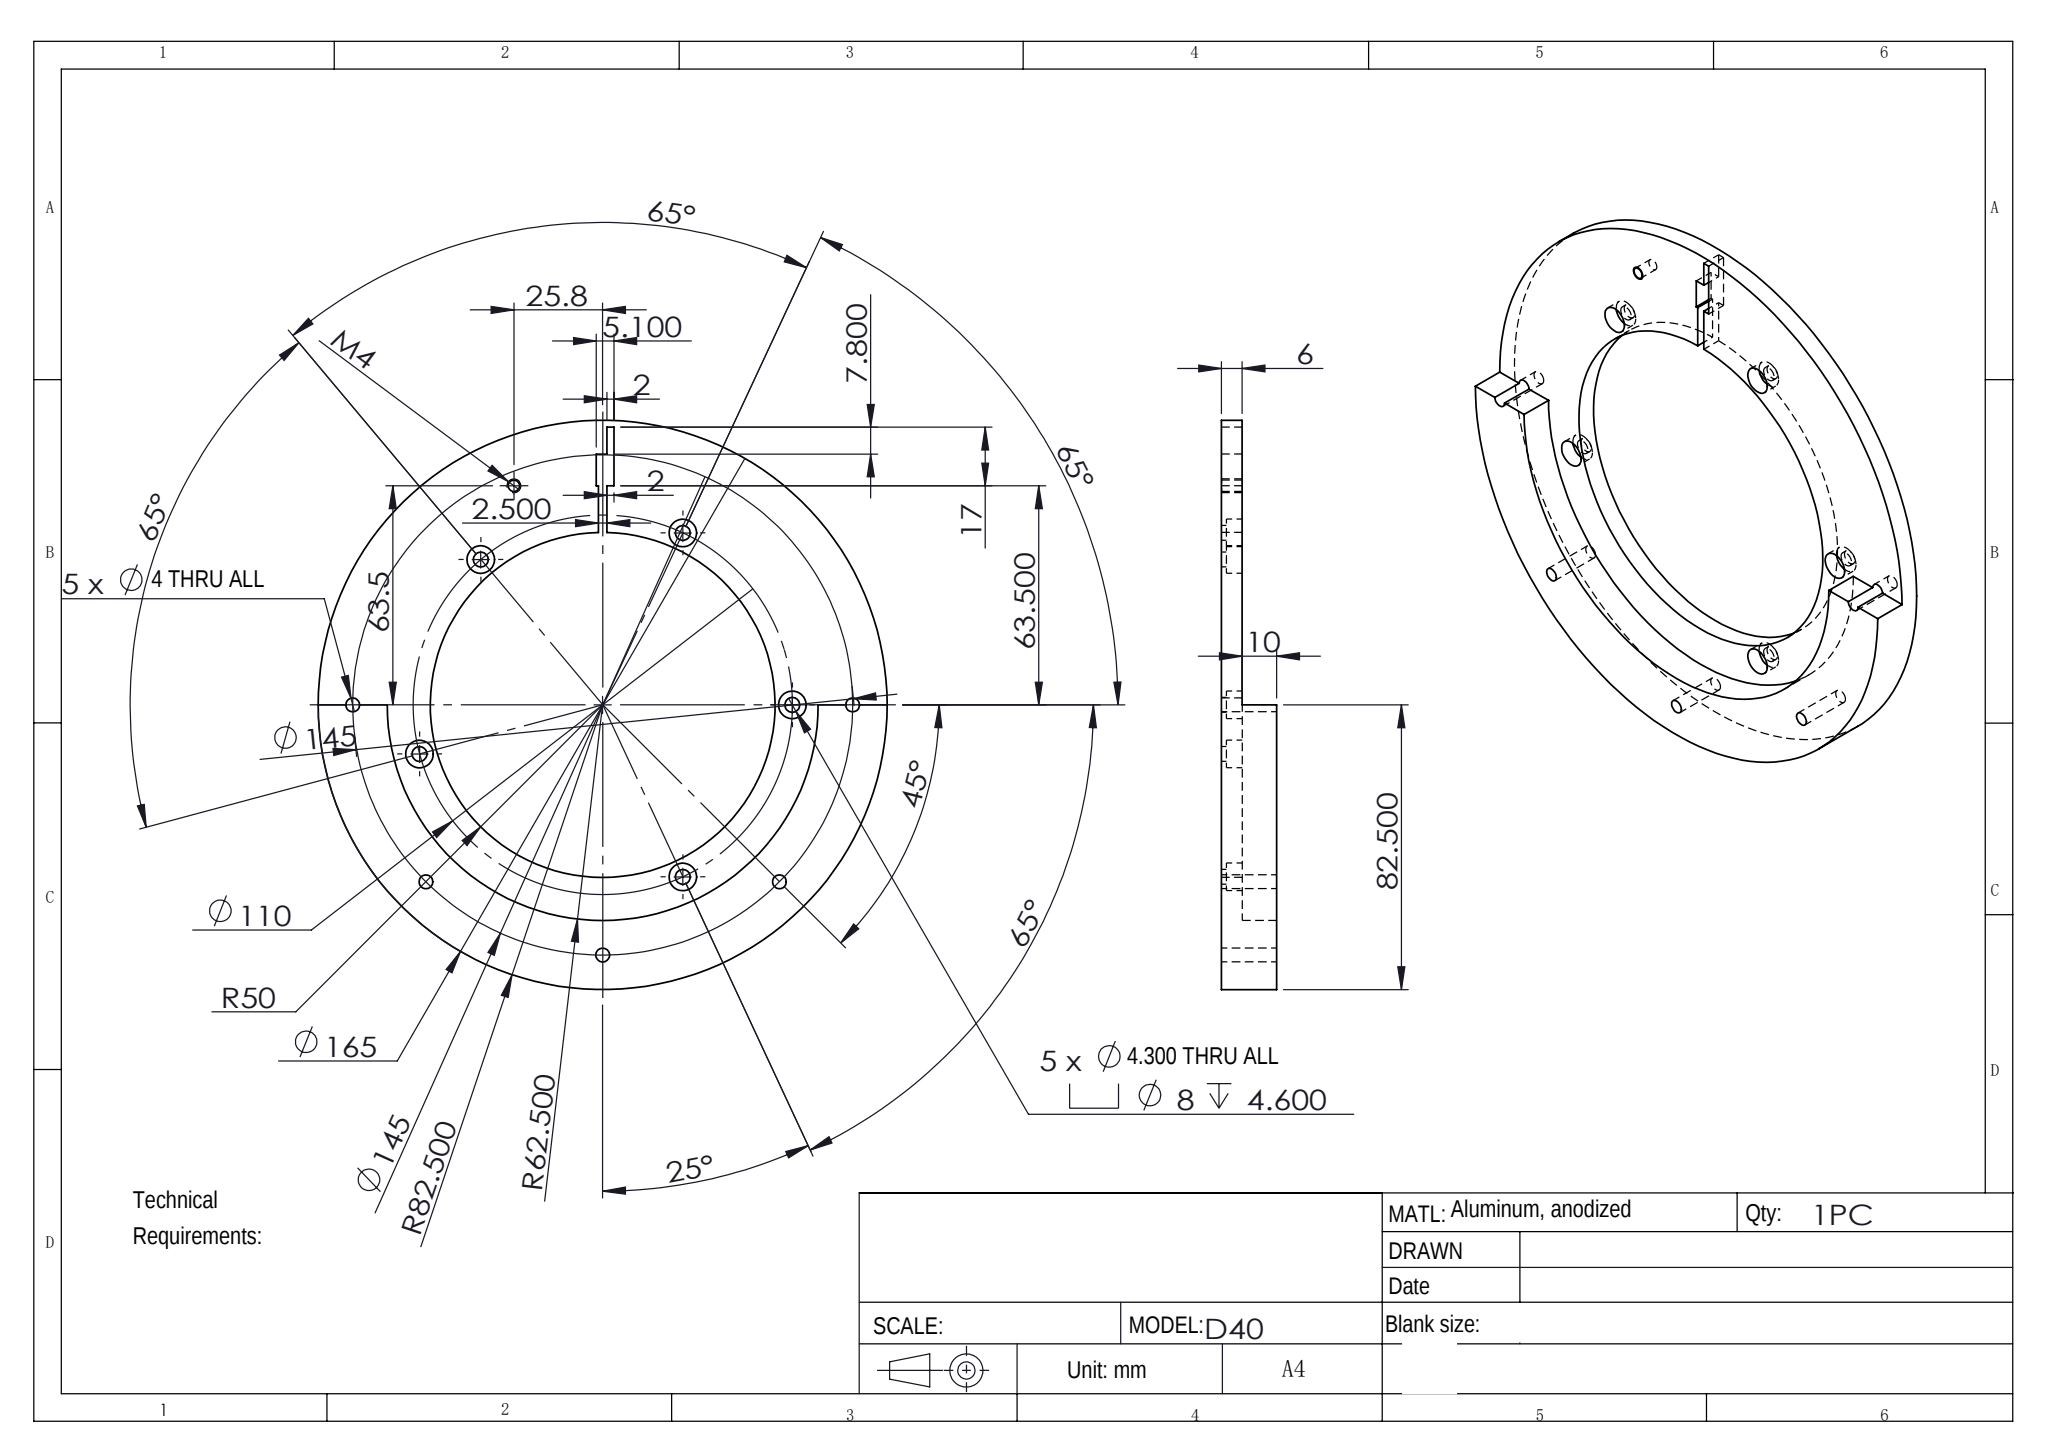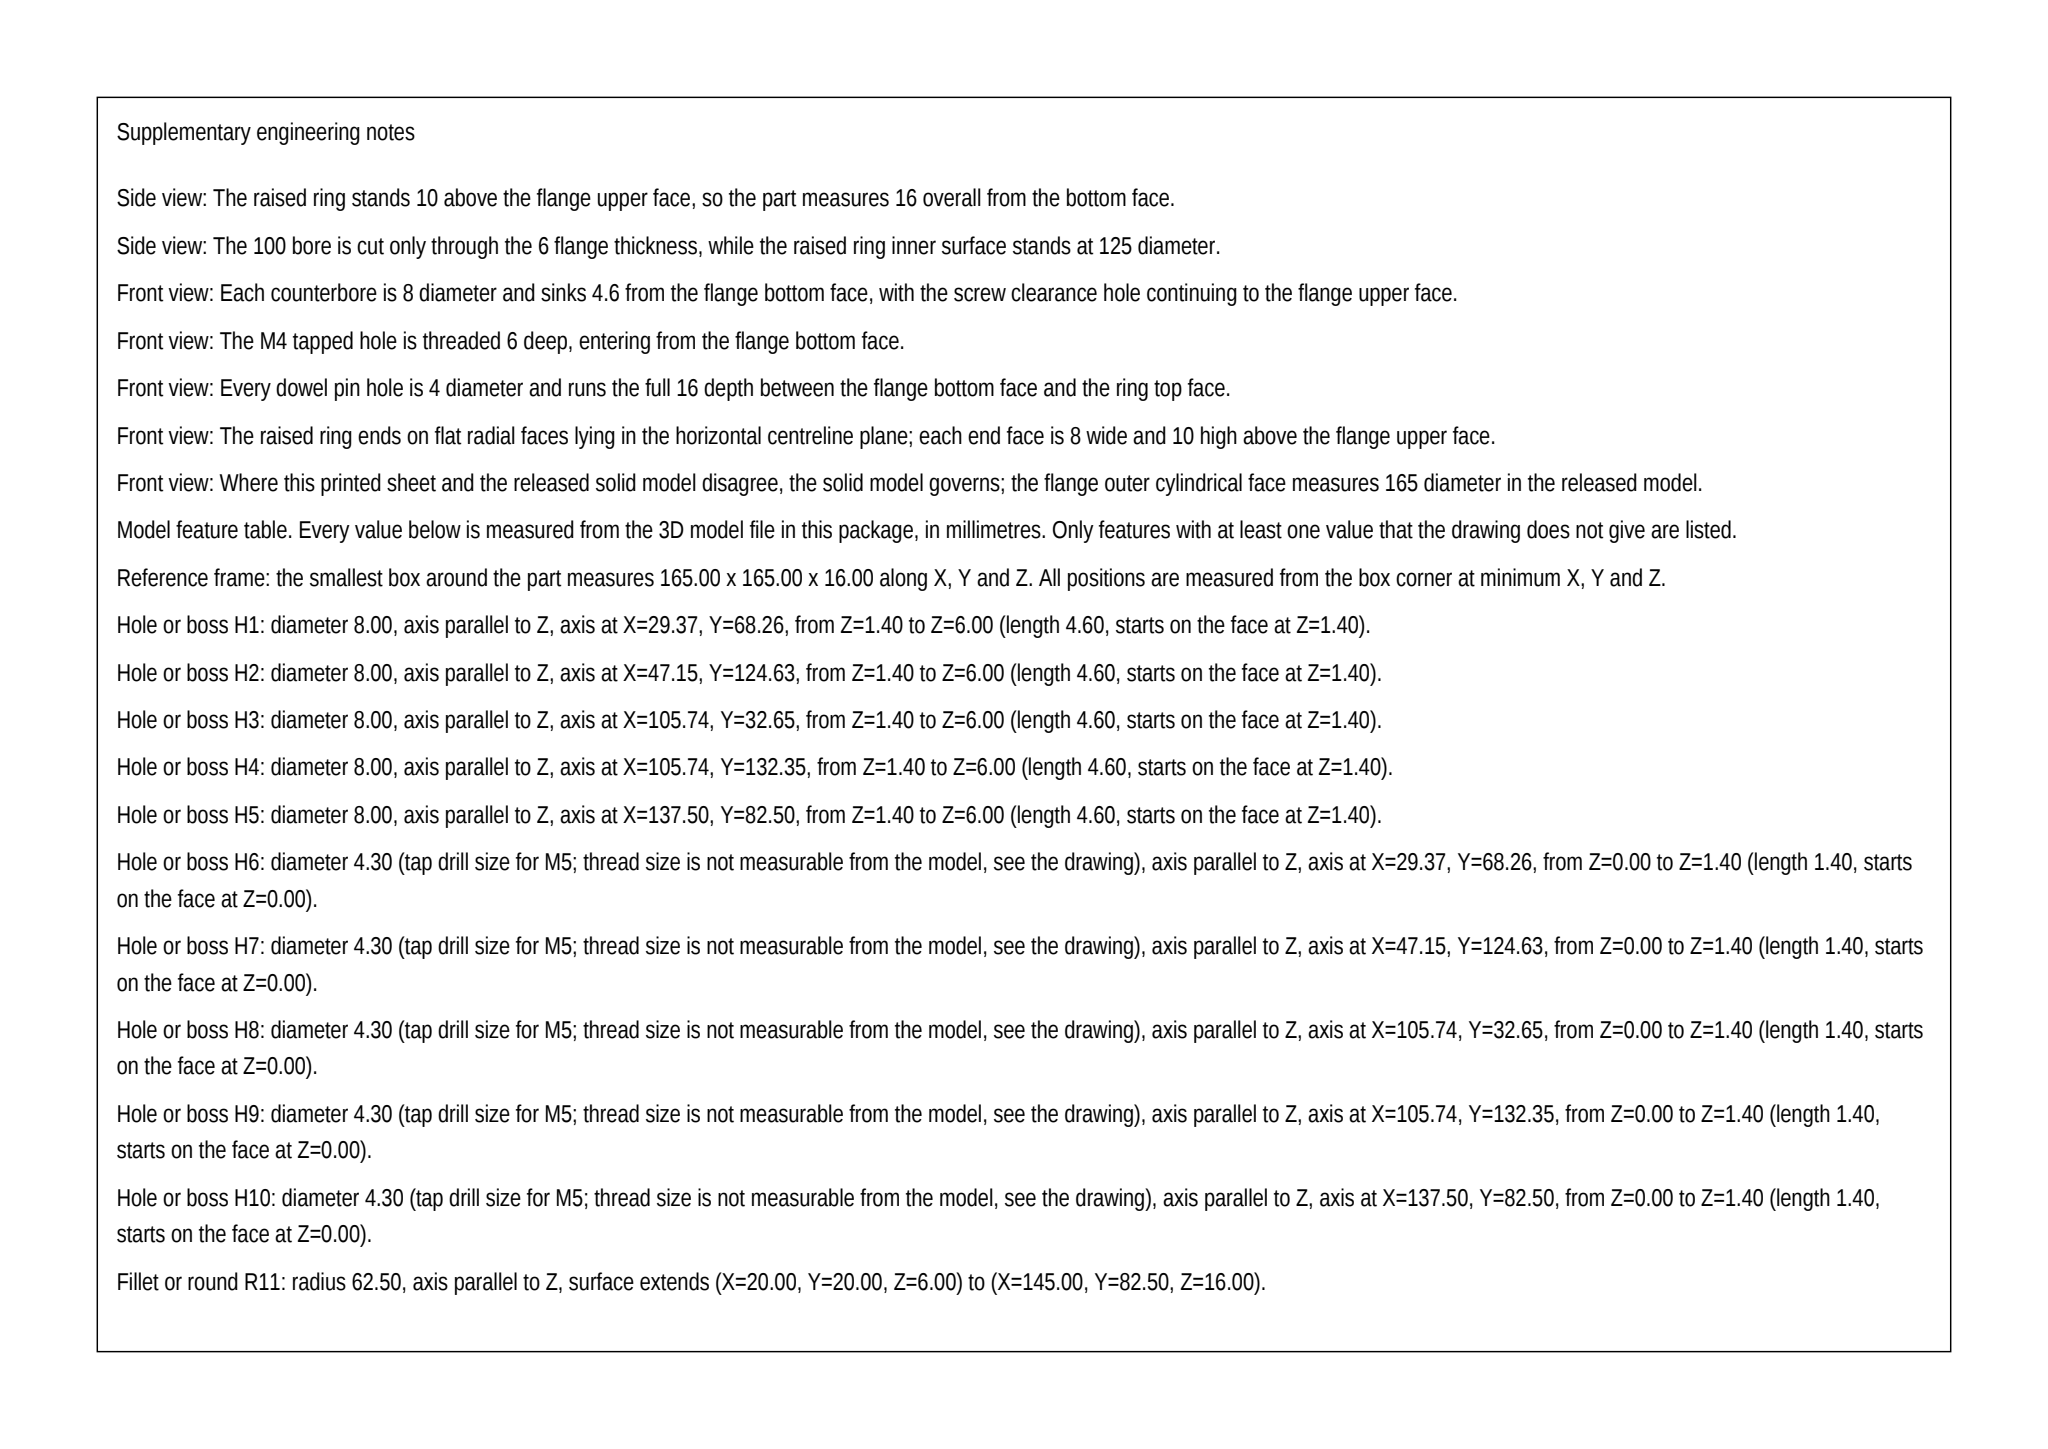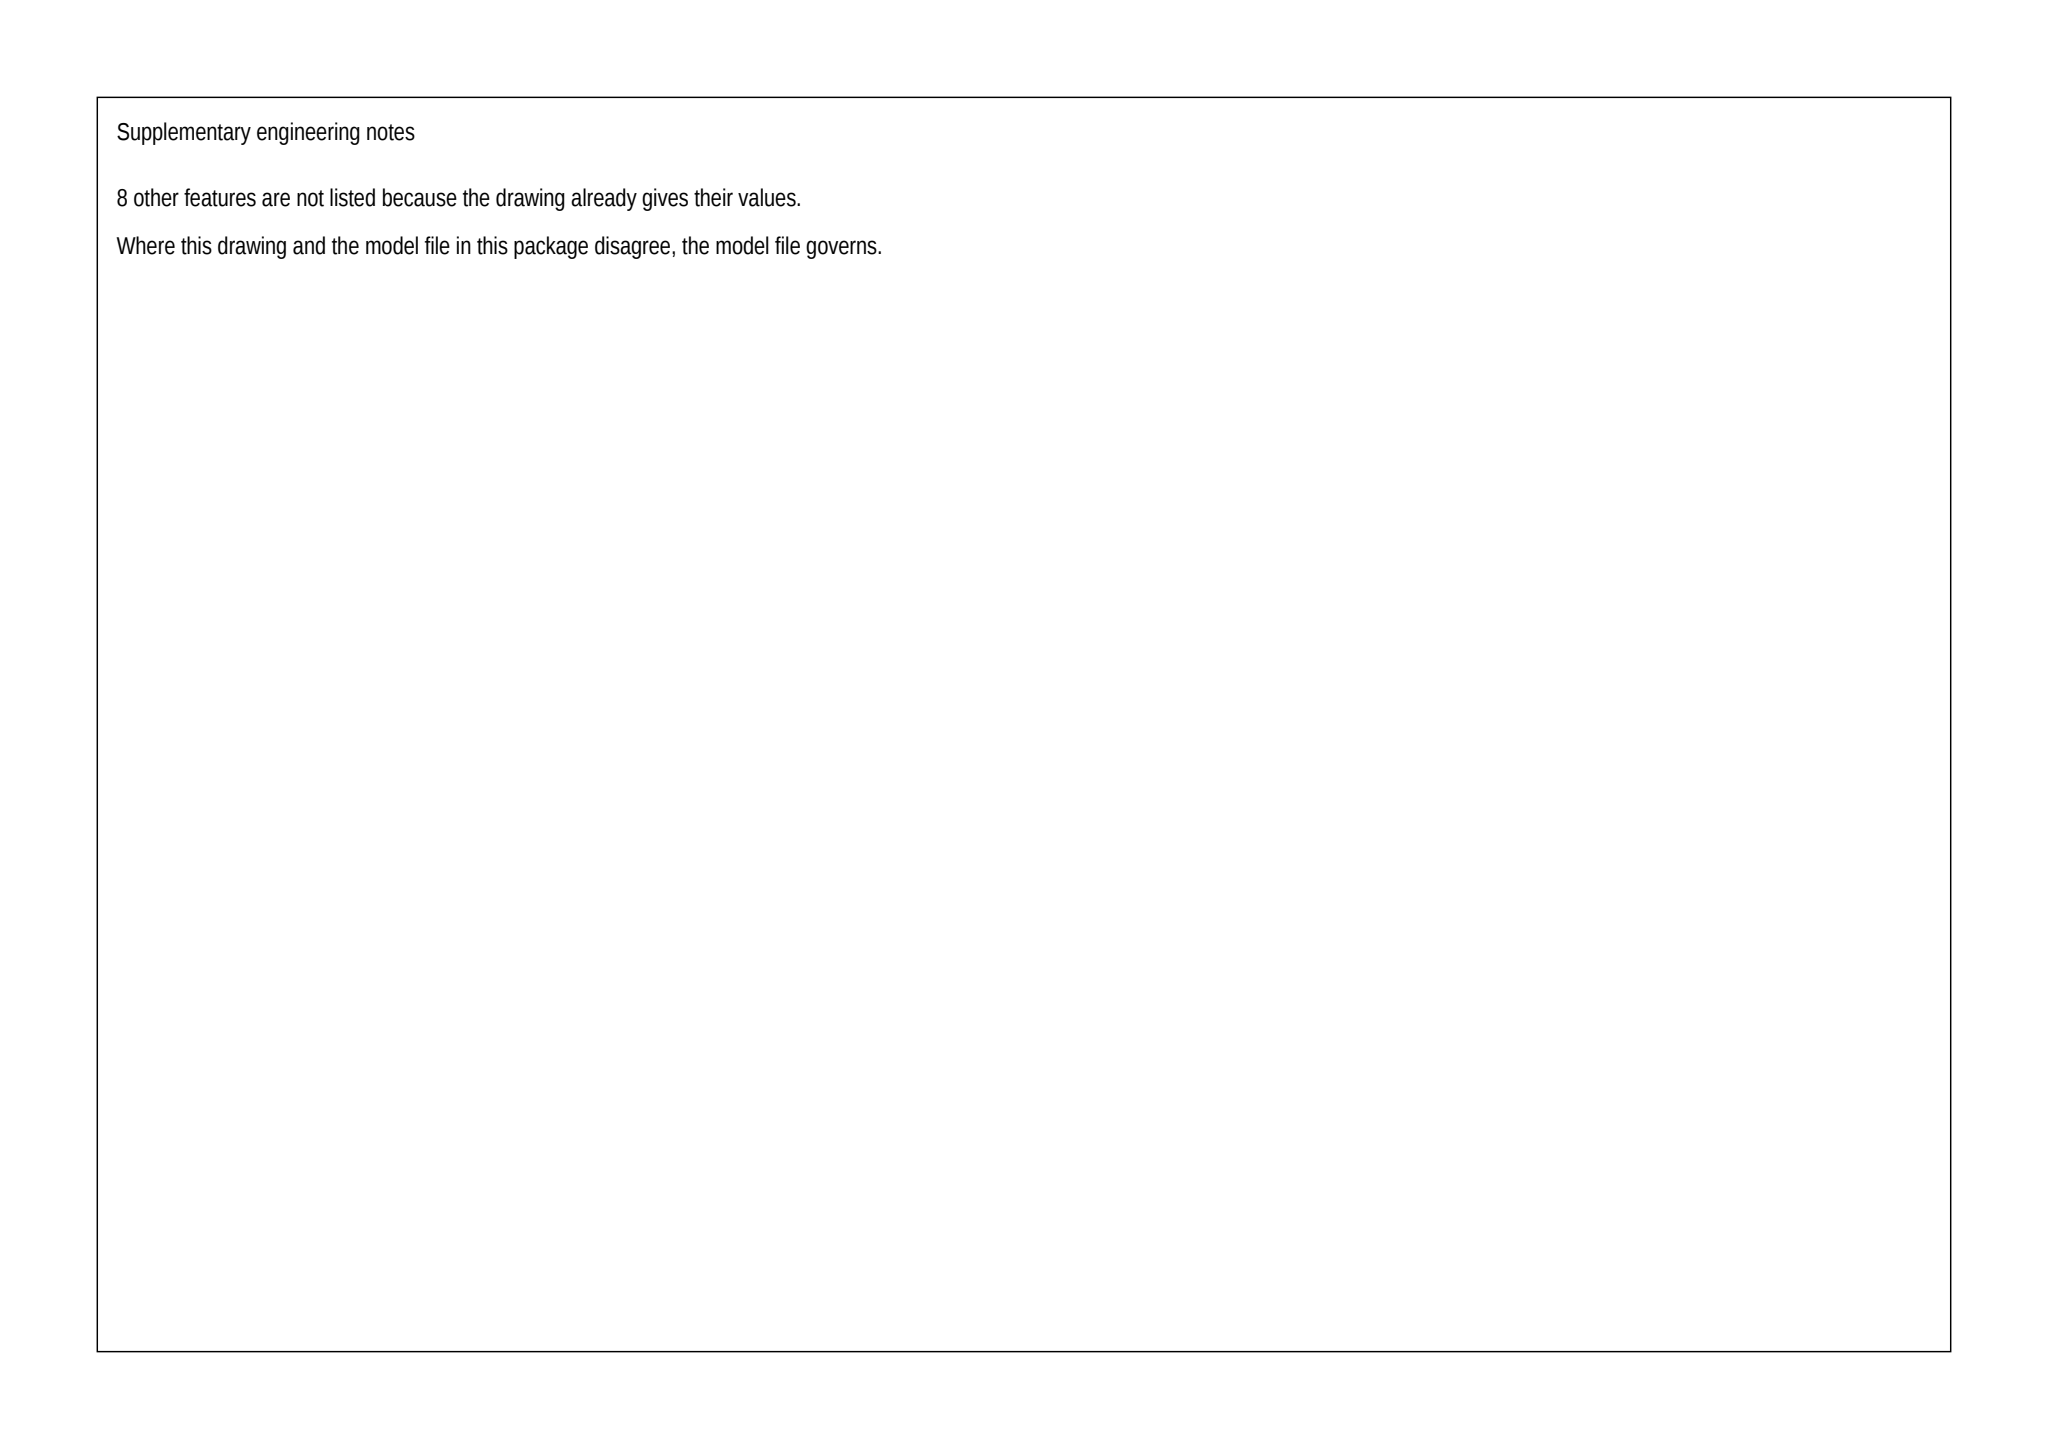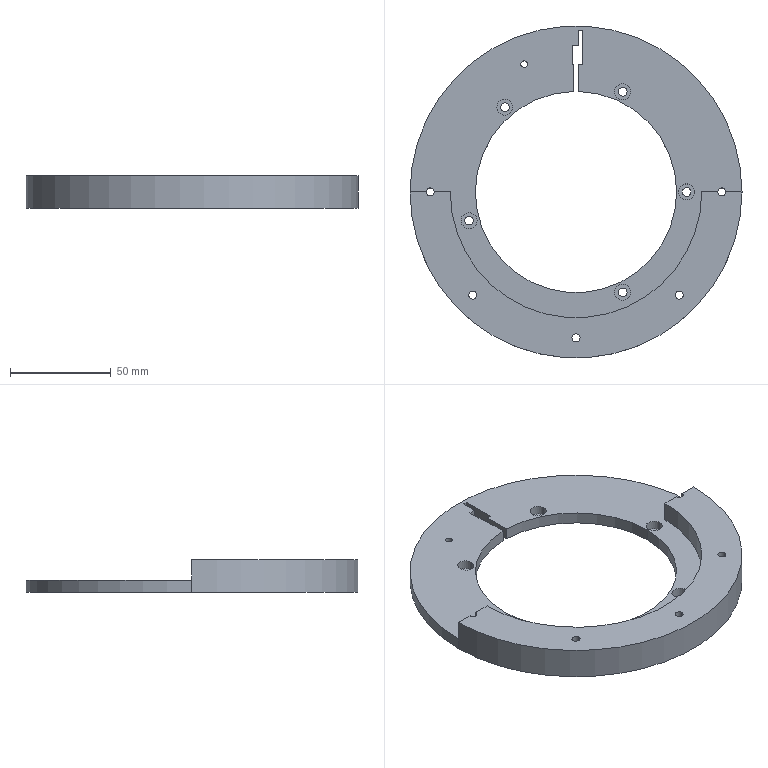Part | SolidWorks | mm | material Aluminum, Anodized | 1 solid | 59 faces | box 165 x 165 x 16 mm | volume 123958 mm3 | cylinder 38 | plane 21 | commonest cylinder face diameters 4 x10 8 x10 4.3 x10 100 x3 3.3 x2 165 x2 125 x1
build123d program:
from build123d import *

# Parameters (mm, degrees)
SKETCH1_R                                            = 82.5
SKETCH1_R_2                                          = 50
BOSS_EXTRUDE1_DEPTH                                  = 6
CUT_EXTRUDE2_DEPTH                                   = 10
SKETCH4_R                                            = 1
CUT_EXTRUDE3_DEPTH                                   = 10
HOLE_SIZE_ACCORDING_TO_HEX_SOCKET_HEAD_C_D           = 4.3
HOLE_SIZE_ACCORDING_TO_HEX_SOCKET_HEAD_C_CBORE_D     = 8
HOLE_SIZE_ACCORDING_TO_HEX_SOCKET_HEAD_C_CBORE_DEPTH = 4.6
M4_TAPPED_HOLE1_D                                    = 3.3
M4_TAPPED_HOLE1_DEPTH                                = 10.1
M4_TAPPED_HOLE1_TIP                                  = 0.9914
BOSS_EXTRUDE2_DEPTH                                  = 10
F_4_0MM_DOWEL_PIN_HOLE_1_D                           = 4


with BuildPart() as part:
    # Sketch1 → Boss-Extrude1 (new body)
    with BuildSketch(Plane.XY):
        Circle(SKETCH1_R)
        Circle(SKETCH1_R_2, mode=Mode.SUBTRACT)
    extrude(amount=BOSS_EXTRUDE1_DEPTH)

    # Sketch3 → Cut-Extrude2 (cut)
    with BuildSketch(Plane.XY.offset(6)):
        Polygon((1.25, 63.5), (1.25, 48.55), (-1.25, 48.55), (-1.25, 63.5), (-1.85, 63.5), (-1.85, 72.7), (1.25, 72.7), (1.25, 80.5), (3.25, 80.5), (3.25, 63.5), align=None)
    extrude(amount=-CUT_EXTRUDE2_DEPTH, mode=Mode.SUBTRACT)

    # Sketch4 → Cut-Extrude3 (cut)
    with BuildSketch(Plane(origin=(0, 0, 0), x_dir=(-1, 0, 0), z_dir=(0, 0, -1))):
        with Locations((25.75, 63.5)):
            Circle(SKETCH4_R)
    extrude(amount=-CUT_EXTRUDE3_DEPTH, mode=Mode.SUBTRACT)

    # Hole Size According to Hex Socket Head C (through all)
    with Locations(Plane.XY.offset(6)):
        with Locations((-53.126, -14.235), (23.244, -49.847), (55, 0), (-35.353, 42.132), (23.244, 49.847)):
            CounterBoreHole(HOLE_SIZE_ACCORDING_TO_HEX_SOCKET_HEAD_C_D / 2, HOLE_SIZE_ACCORDING_TO_HEX_SOCKET_HEAD_C_CBORE_D / 2, HOLE_SIZE_ACCORDING_TO_HEX_SOCKET_HEAD_C_CBORE_DEPTH)

    # M4 Tapped Hole1
    with Locations(Plane.XY.offset(6)):
        with Locations((-25.75, 63.5)):
            Hole(M4_TAPPED_HOLE1_D / 2, depth=M4_TAPPED_HOLE1_DEPTH)
            with Locations((0, 0, -(M4_TAPPED_HOLE1_DEPTH + M4_TAPPED_HOLE1_TIP / 2))):  # 118° drill point
                Cone(0, M4_TAPPED_HOLE1_D / 2, M4_TAPPED_HOLE1_TIP, mode=Mode.SUBTRACT)

    # Sketch9 → Boss-Extrude2 (add)
    with BuildSketch(Plane.XY.offset(6)):
        with BuildLine():
            Line((-82.5, 0), (-62.5, 0))
            ThreePointArc((-62.5, 0), (0, -62.5), (62.5, 0))
            Line((62.5, 0), (82.5, 0))
            ThreePointArc((82.5, 0), (0, -82.5), (-82.5, 0))
        make_face()
    extrude(amount=BOSS_EXTRUDE2_DEPTH)

    # 4.0mm Dowel Pin Hole 1 (through all)
    with Locations(Plane.XY.offset(16)):
        with Locations((72.5, 0), (-72.5, 0), (-51.265, -51.265), (0, -72.5), (51.265, -51.265)):
            Hole(F_4_0MM_DOWEL_PIN_HOLE_1_D / 2)


solid = part.part